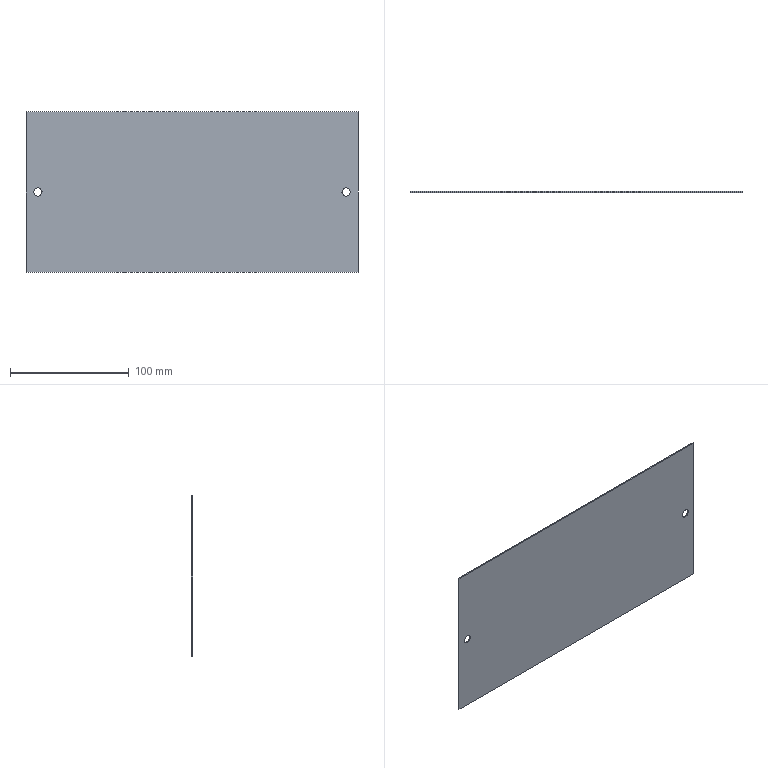Component | SolidWorks | TopCoverCableHoleBlankingPlate-1 | 1 solid | 10 faces | volume 33951 mm3 | plane 6 | cylinder 4 | commonest cylinder face diameters 7 x4